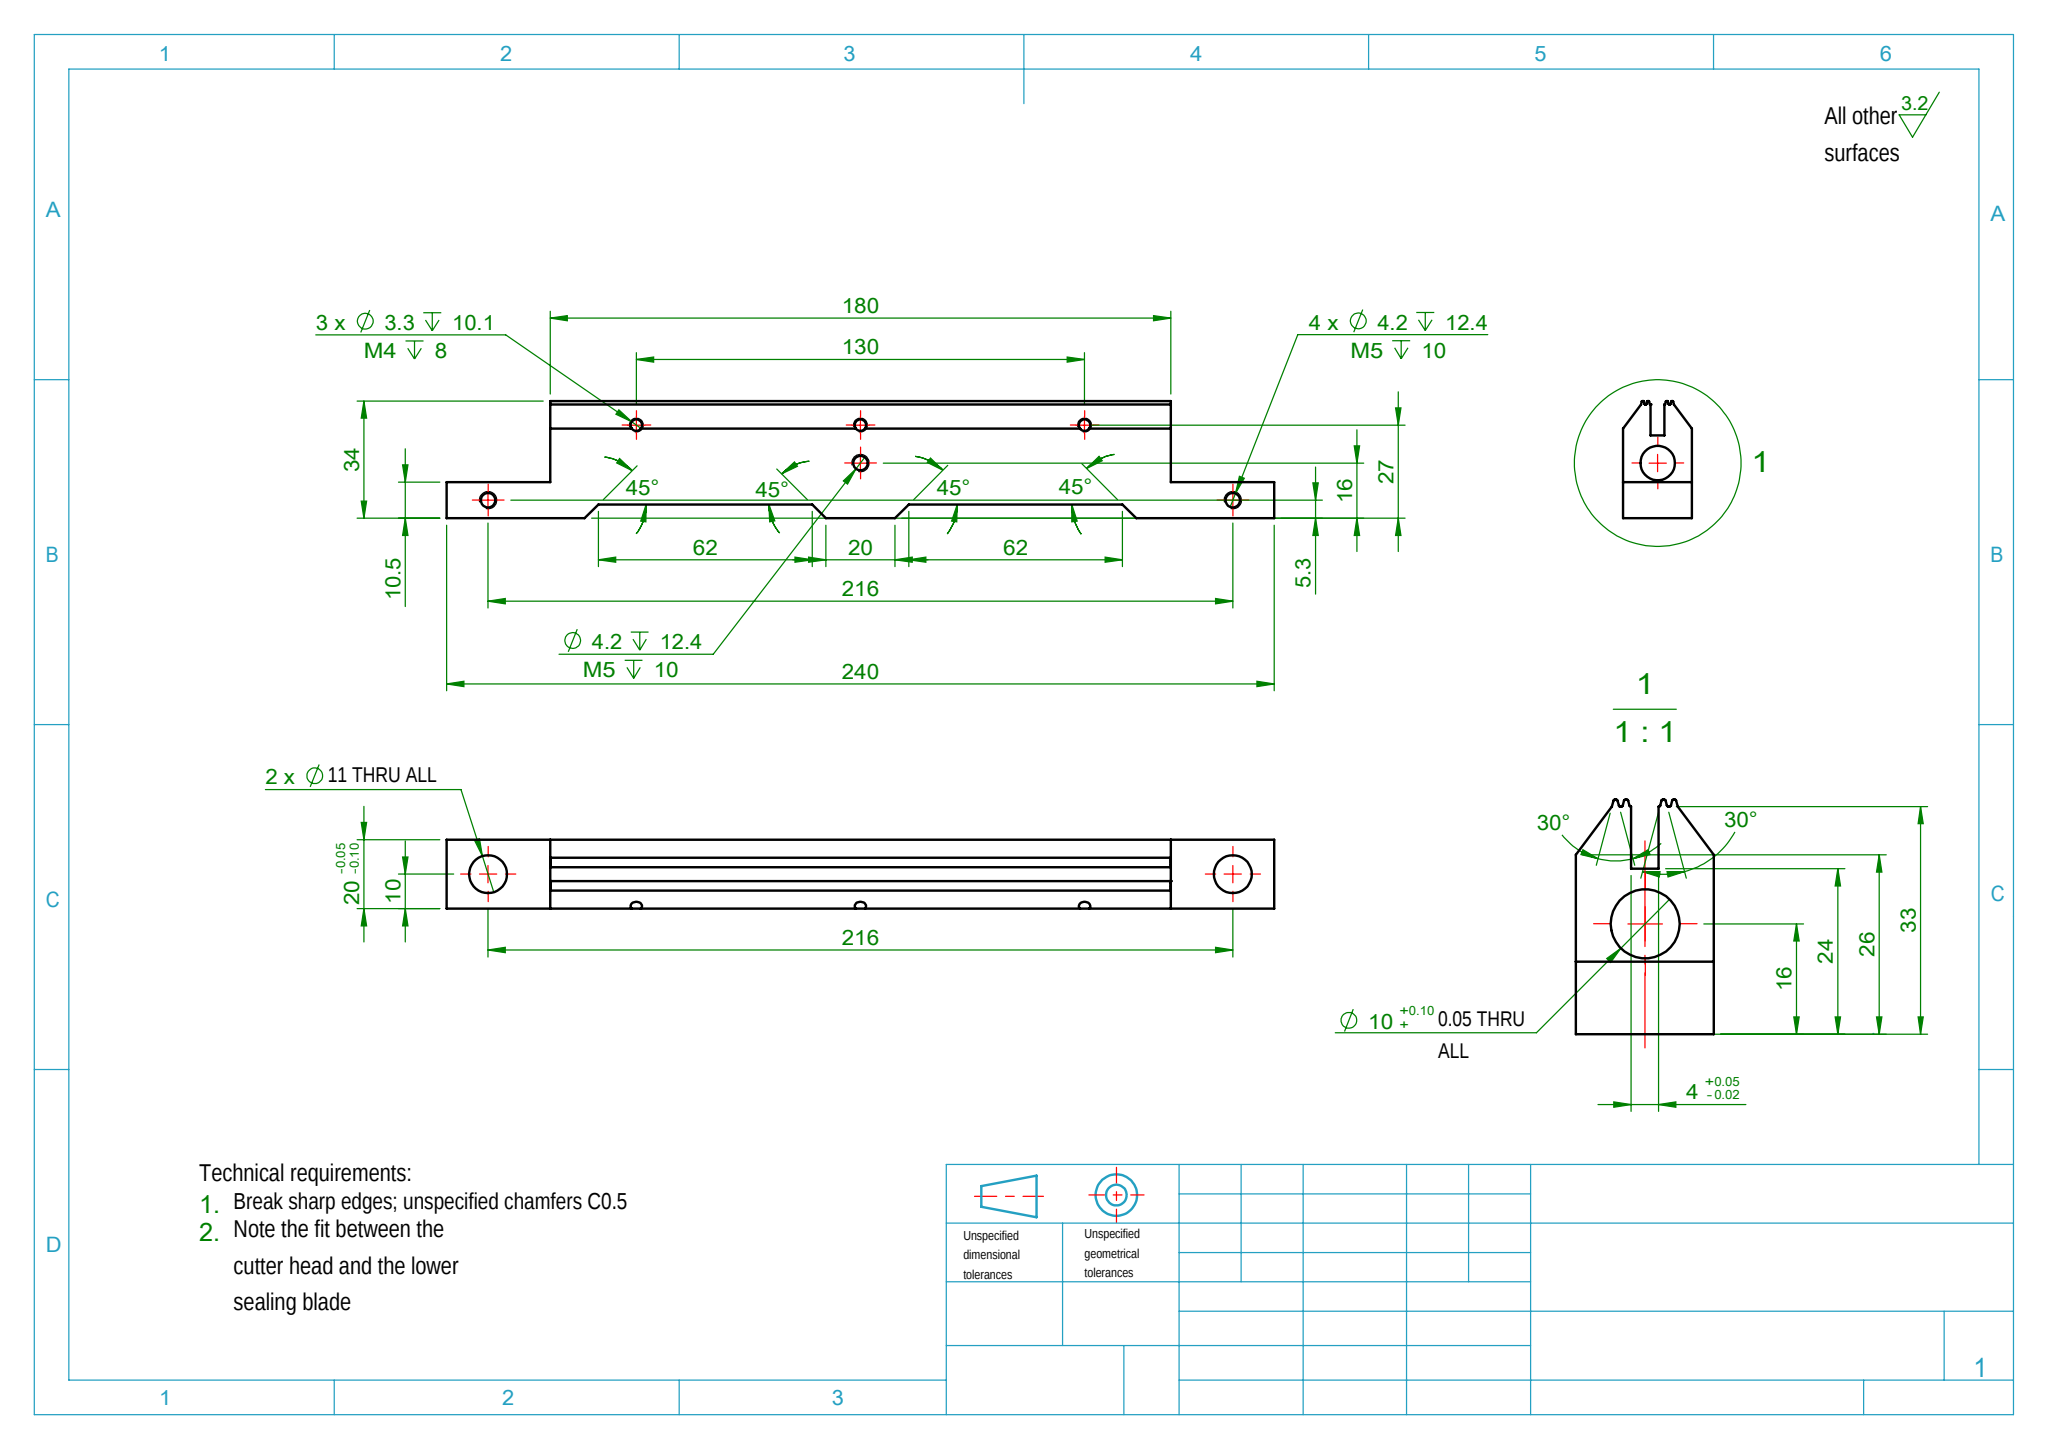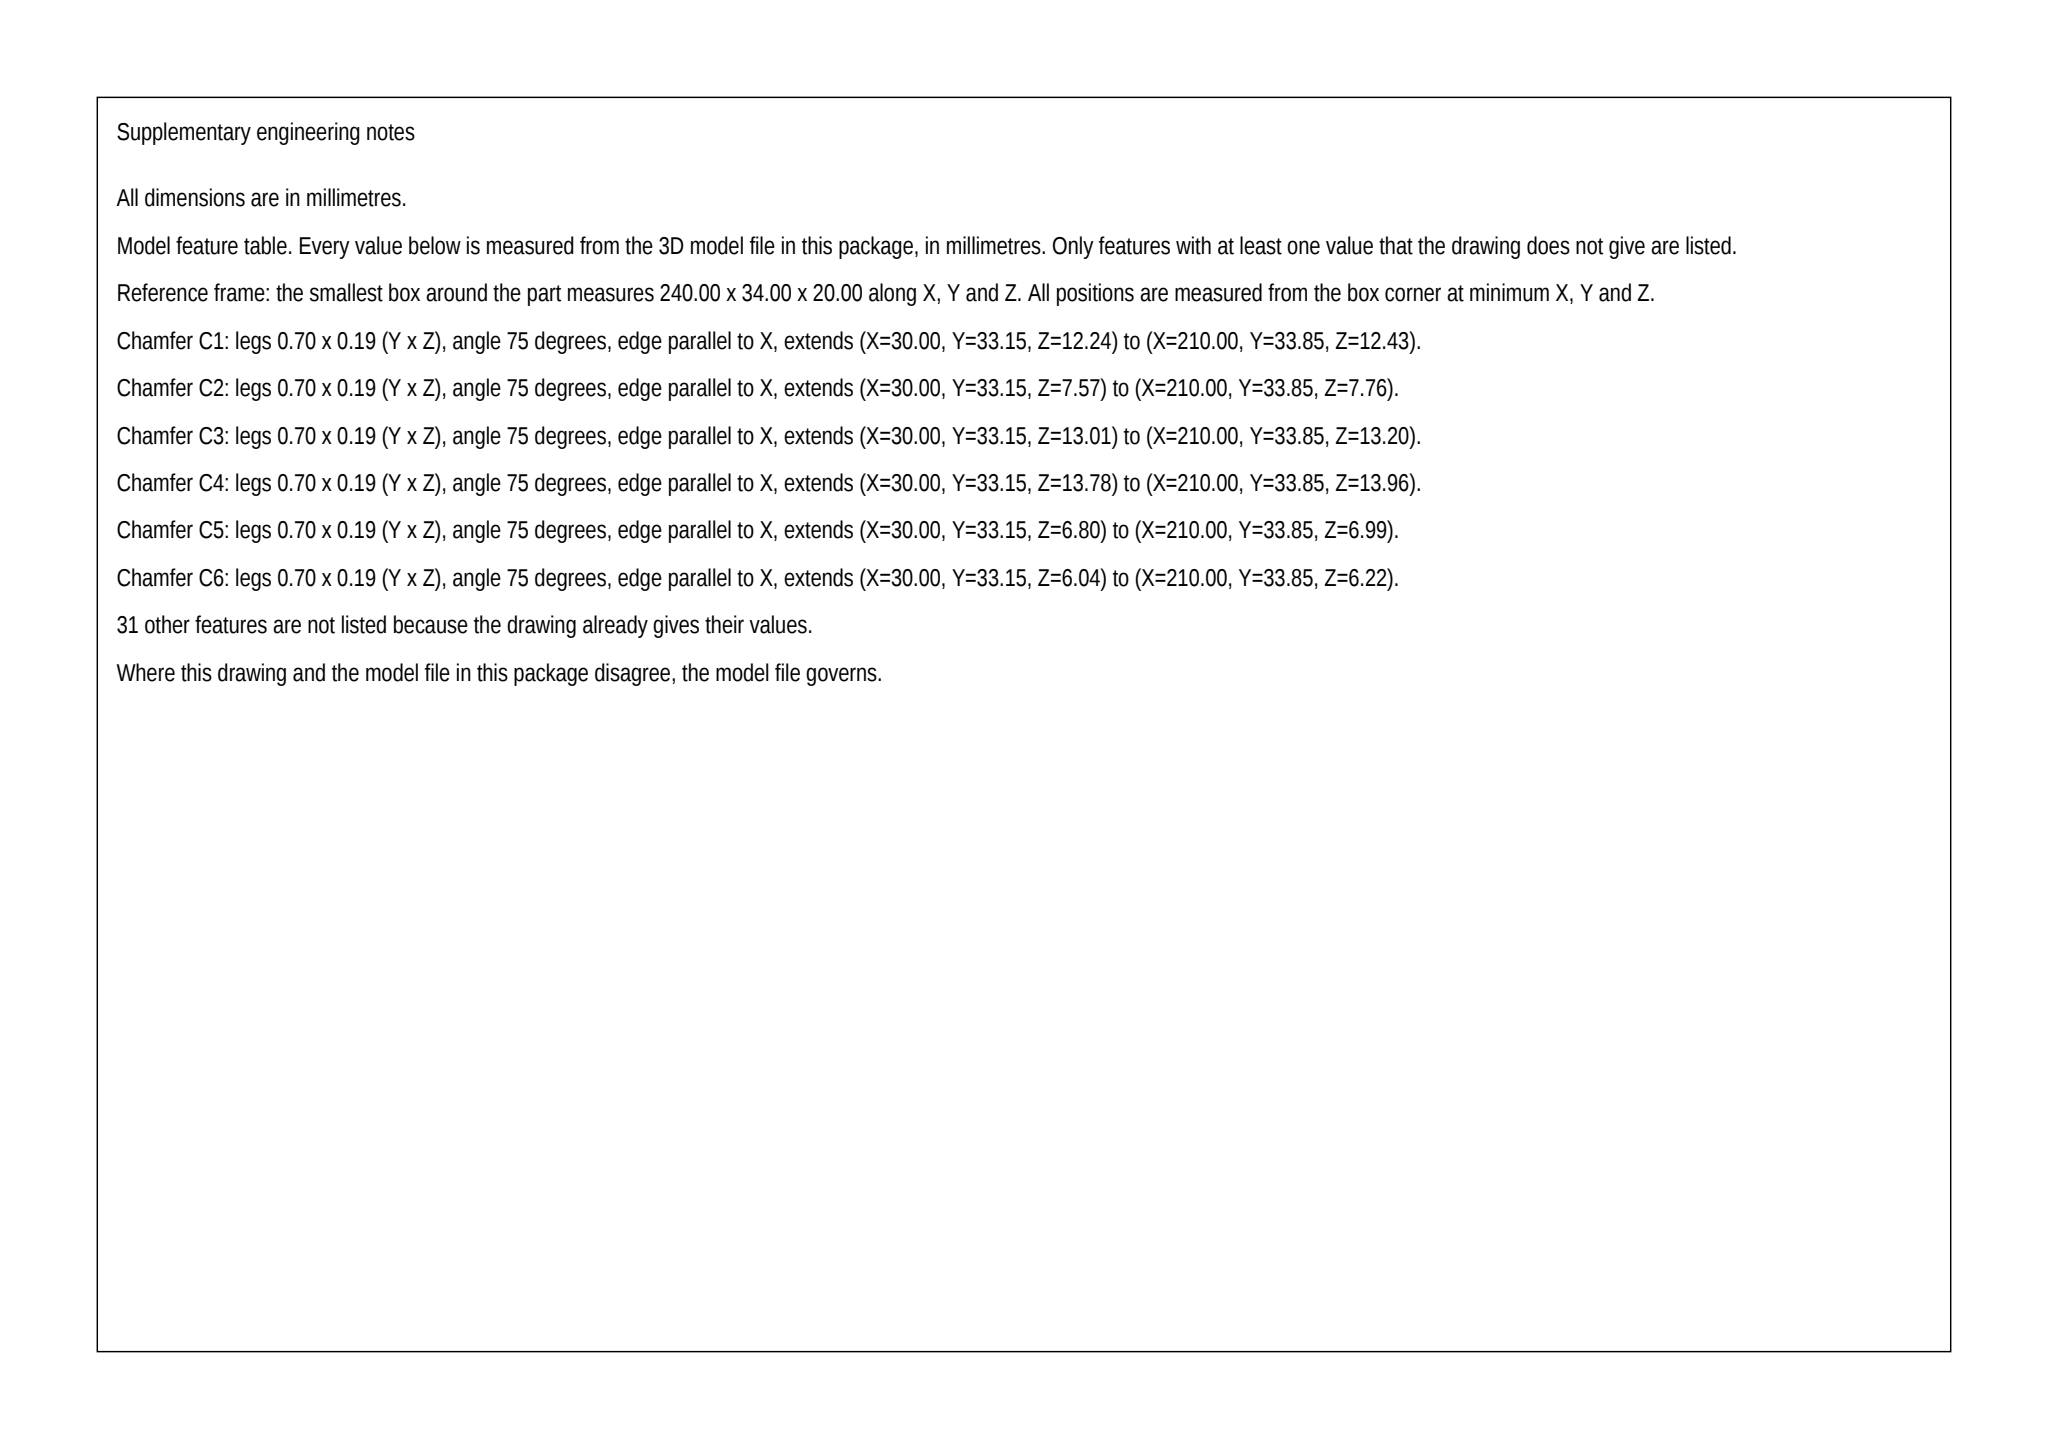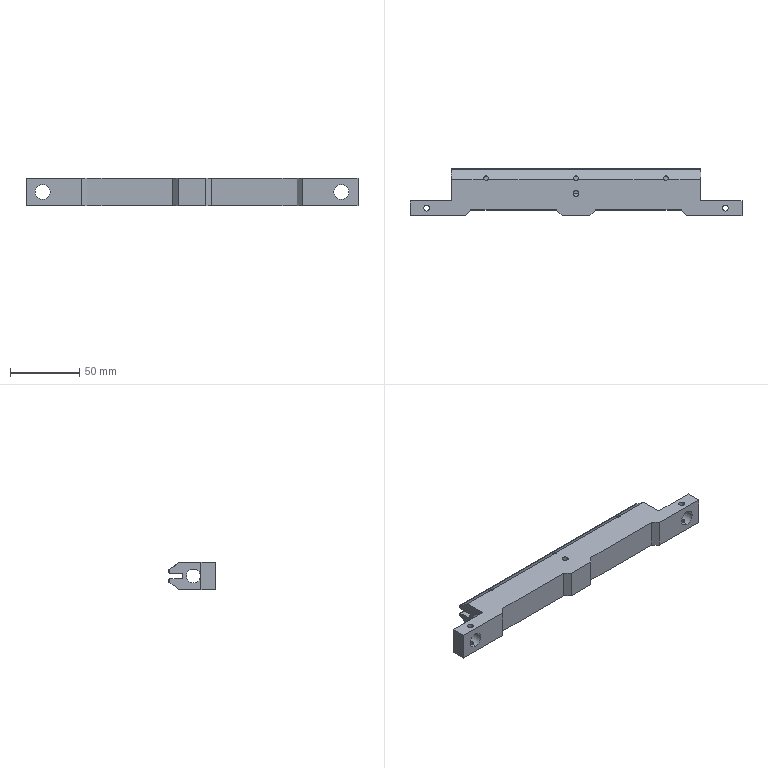Part | SolidWorks | mm | 1 solid | 74 faces | box 240 x 34 x 20 mm | volume 91680 mm3 | plane 38 | cylinder 36 | commonest cylinder face diameters 0.4 x14 4.2 x10 3.3 x6 11 x4 10 x2
Drawing notes:
All dimensions in millimetres. | from the solid: STEP header/model units: mm (bbox_xyz 240.0 x 34.0 x 20.0 mm)
3X Ø3.3 DP 10.1, M4 DP 8, axes parallel to Z (normal to the 20 wide face), located X = 55, 120 and 185 from the left end face (X0) and Y = 27 from the bottom face (Y0). | from the solid: cylinders 3.3 dia, axis z, pos [55,27], [120,27], [185,27], lengths 8.0/7.25
1X Ø4.2 DP 12.4, M5 DP 10 in upper body, axis parallel to Z, located X = 120 from the left end face (X0), Y = 16 from the bottom face (Y0). | from the solid: cylinder 4.2 dia, axis z, pos [120.0, 16.0], length 5.41, count 2
4X Ø4.2 DP 12.4, M5 DP 10: two at X = 12 and two at X = 228 from the left end face (X0), all at Y = 5.25 from the bottom face (Y0). | from the solid: cylinders 4.2 dia, axis z, pos [12.0,5.25] count 4 and [228.0,5.25] count 4
2X Ø11 holes, axes parallel to Y, located X = 12 and X = 228 from the left end face (X0) and Z = 10 from the Z0 face; depth 10.5 from the Y0 face. | from the solid: cylinders 11.0 dia, axis y, pos [12.0,-,10.0] and [228.0,-,10.0], length 10.5
Ø10 +0.10/+0.05 bore through full length, axis parallel to X, located Y = 16 from the bottom face (Y0) and Z = 10.05 from the Z0 face (20 thickness); bore length 180. | from the solid: cylinder 10.0 dia, axis x, pos [-,16.0,10.05], length 180.0
Stepped body end faces: steps at X = 30 and X = 210 from the left end face (X0); overall length 240. | from the solid: axis_planes x = 0.0, 30.0, 210.0, 240.0; bbox_xyz X = 240.0
Underside relief flat lies at Y = 4 from the bottom face (Y0); lower body faces at Y = 10.5 and Y = 24 from Y0. | from the solid: axis_planes y = 4.0 (count 2), y = 10.5 (count 2), y = 24.0
Serration tip/root rounds: R0.2 (Ø0.4) full 180 length, axes parallel to X. Row at Y = 33.2 from Y0 at Z = 6.42, 6.61, 7.95, 12.05, 13.39, 13.58; row at Y = 33.8 from Y0 at Z = 5.65, 5.84, 7.19, 7.38, 12.62, 12.81, 14.16, 14.35 (Z from the Z0 face). | from the solid: cylinders 0.4 dia, axis x, pos y=33.2 at z=6.42/6.61/7.95/12.05/13.39/13.58 and y=33.8 at z=5.65/5.84/7.19/7.38/12.62/12.81/14.16/14.35, each length 180.0
Blade/tooth crest faces at Y = 33 and Y = 34 from the bottom face (Y0); overall height 34. | from the solid: axis_planes y = 33.0 (count 4), y = 34.0 (count 4); bbox_xyz Y = 34.0
build123d program:
from build123d import *

# Parameters (mm, degrees)
BOSS_EXTRUDE1_DEPTH        = 20
F_10_0_10_DIAMETER_HOLE1_D = 10
M10_CLEARANCE_HOLE1_D      = 11
CUT_EXTRUDE1_DEPTH         = 213.255
FILLET1_R                  = 0.2
M4_TAPPED_HOLE1_D          = 3.3
M4_TAPPED_HOLE1_DEPTH      = 10.1
M4_TAPPED_HOLE1_TIP        = 0.9914
M5_TAPPED_HOLE1_D          = 4.2
M5_TAPPED_HOLE1_DEPTH      = 12.4
M5_TAPPED_HOLE1_TIP        = 1.262
M5_TAPPED_HOLE2_AT_2_COUNT = 2
M5_TAPPED_HOLE2_AT_2_PITCH = 216
CUT_EXTRUDE2_DEPTH         = 242.976


with BuildPart() as part:
    # Sketch1 → Boss-Extrude1 (new body)
    with BuildSketch(Plane.XY):
        Polygon((0, 0), (30, 0), (30, 23.5), (210, 23.5), (210, 0), (240, 0), (240, -10.5), (0, -10.5), align=None)
    extrude(amount=BOSS_EXTRUDE1_DEPTH)

    # 10.0 _10_ Diameter Hole1 (through all)
    with Locations(Plane(origin=(210, 0, 0), x_dir=(0, 0, -1), z_dir=(1, 0, 0))):
        with Locations((-10.053, 5.5)):
            Hole(F_10_0_10_DIAMETER_HOLE1_D / 2)

    # M10 Clearance Hole1 (through all)
    with Locations(Plane(origin=(0, 0, 0), x_dir=(1, 0, 0), z_dir=(0, 1, 0))):
        with Locations((12, -10), (228, -10)):
            Hole(M10_CLEARANCE_HOLE1_D / 2)

    # Sketch7 → Cut-Extrude1 (cut, through all)
    with BuildSketch(Plane.ZY.offset(-30)):
        Polygon((8, 13.5), (12, 13.5), (12, 22.5), (12.2, 22.5), (12.468, 23.5), (12.968, 23.5), (13.236, 22.5), (13.736, 22.5), (14.004, 23.5), (14.504, 23.5), (14.772, 22.5), (20, 15.5), (20, 25.5), (0, 25.5), (0, 15.5), (5.228, 22.5), (5.496, 23.5), (5.996, 23.5), (6.264, 22.5), (6.764, 22.5), (7.032, 23.5), (7.532, 23.5), (7.8, 22.5), (8, 22.5), align=None)
    extrude(amount=-CUT_EXTRUDE1_DEPTH, mode=Mode.SUBTRACT)

    # Fillet1
    fillet1_edges = [part.edges().sort_by_distance(p)[0] for p in [
        (120, 22.5, 7.8),
        (120, 23.5, 7.532),
        (120, 23.5, 7.032),
        (120, 22.5, 6.764),
        (120, 22.5, 6.264),
        (120, 23.5, 5.996),
        (120, 23.5, 5.496),
        (120, 23.5, 14.504),
        (120, 23.5, 14.004),
        (120, 22.5, 13.736),
        (120, 22.5, 13.236),
        (120, 23.5, 12.968),
        (120, 23.5, 12.468),
        (120, 22.5, 12.2),
    ]]
    fillet(fillet1_edges, radius=FILLET1_R)

    # M4 Tapped Hole1
    with Locations(Plane.XY.offset(20)):
        with Locations((55, 16.5), (120, 16.5), (185, 16.5)):
            Hole(M4_TAPPED_HOLE1_D / 2, depth=M4_TAPPED_HOLE1_DEPTH)
            with Locations((0, 0, -(M4_TAPPED_HOLE1_DEPTH + M4_TAPPED_HOLE1_TIP / 2))):  # 118° drill point
                Cone(0, M4_TAPPED_HOLE1_D / 2, M4_TAPPED_HOLE1_TIP, mode=Mode.SUBTRACT)

    # M5 Tapped Hole1
    with Locations(Plane.XY.offset(20)):
        with Locations((120, 5.5)):
            Hole(M5_TAPPED_HOLE1_D / 2, depth=M5_TAPPED_HOLE1_DEPTH)
            with Locations((0, 0, -(M5_TAPPED_HOLE1_DEPTH + M5_TAPPED_HOLE1_TIP / 2))):  # 118° drill point
                Cone(0, M5_TAPPED_HOLE1_D / 2, M5_TAPPED_HOLE1_TIP, mode=Mode.SUBTRACT)

    # Sketch13 → M5 Tapped Hole2 (revolve, cut)
    with BuildSketch(Plane(origin=(12, -5.25, 20), x_dir=(0, -1, 0), z_dir=(1, 0, 0))):
        Polygon((0, 0), (0, 13.662), (2.1, 12.4), (2.1, 0), align=None)
    m5_tapped_hole2 = revolve(axis=Axis((12, -5.25, 26.35), (0, 0, -1)), mode=Mode.SUBTRACT)

    # M5 Tapped Hole2 at 2: M5 Tapped Hole2 ×2
    with Locations(*[(i * M5_TAPPED_HOLE2_AT_2_PITCH, 0, 0) for i in range(1, M5_TAPPED_HOLE2_AT_2_COUNT)]):
        add(m5_tapped_hole2, mode=Mode.SUBTRACT)

    # Mirror1: M5 Tapped Hole2 across plane
    add(m5_tapped_hole2.mirror(Plane.XY.offset(10)), mode=Mode.SUBTRACT)

    # Mirror1 copy 1 sketch → Mirror1 copy 1 (revolve, cut)
    with BuildSketch(Plane(origin=(228, -5.25, 0), x_dir=(0, -1, 0), z_dir=(1, 0, 0))):
        Polygon((0, 0), (0, -13.662), (2.1, -12.4), (2.1, 0), align=None)
    revolve(axis=Axis((228, -5.25, -6.35), (0, 0, -1)), mode=Mode.SUBTRACT)

    # Sketch14 → Cut-Extrude2 (cut, through all)
    with BuildSketch(Plane.XY.offset(20)):
        Polygon((40, -10.5), (44, -6.5), (106, -6.5), (110, -10.5), (110, -30.577), (40, -30.577), align=None)
        Polygon((134, -6.5), (196, -6.5), (200, -10.5), (200, -30.577), (130, -30.577), (130, -10.5), align=None)
    extrude(amount=-CUT_EXTRUDE2_DEPTH, mode=Mode.SUBTRACT)


solid = part.part